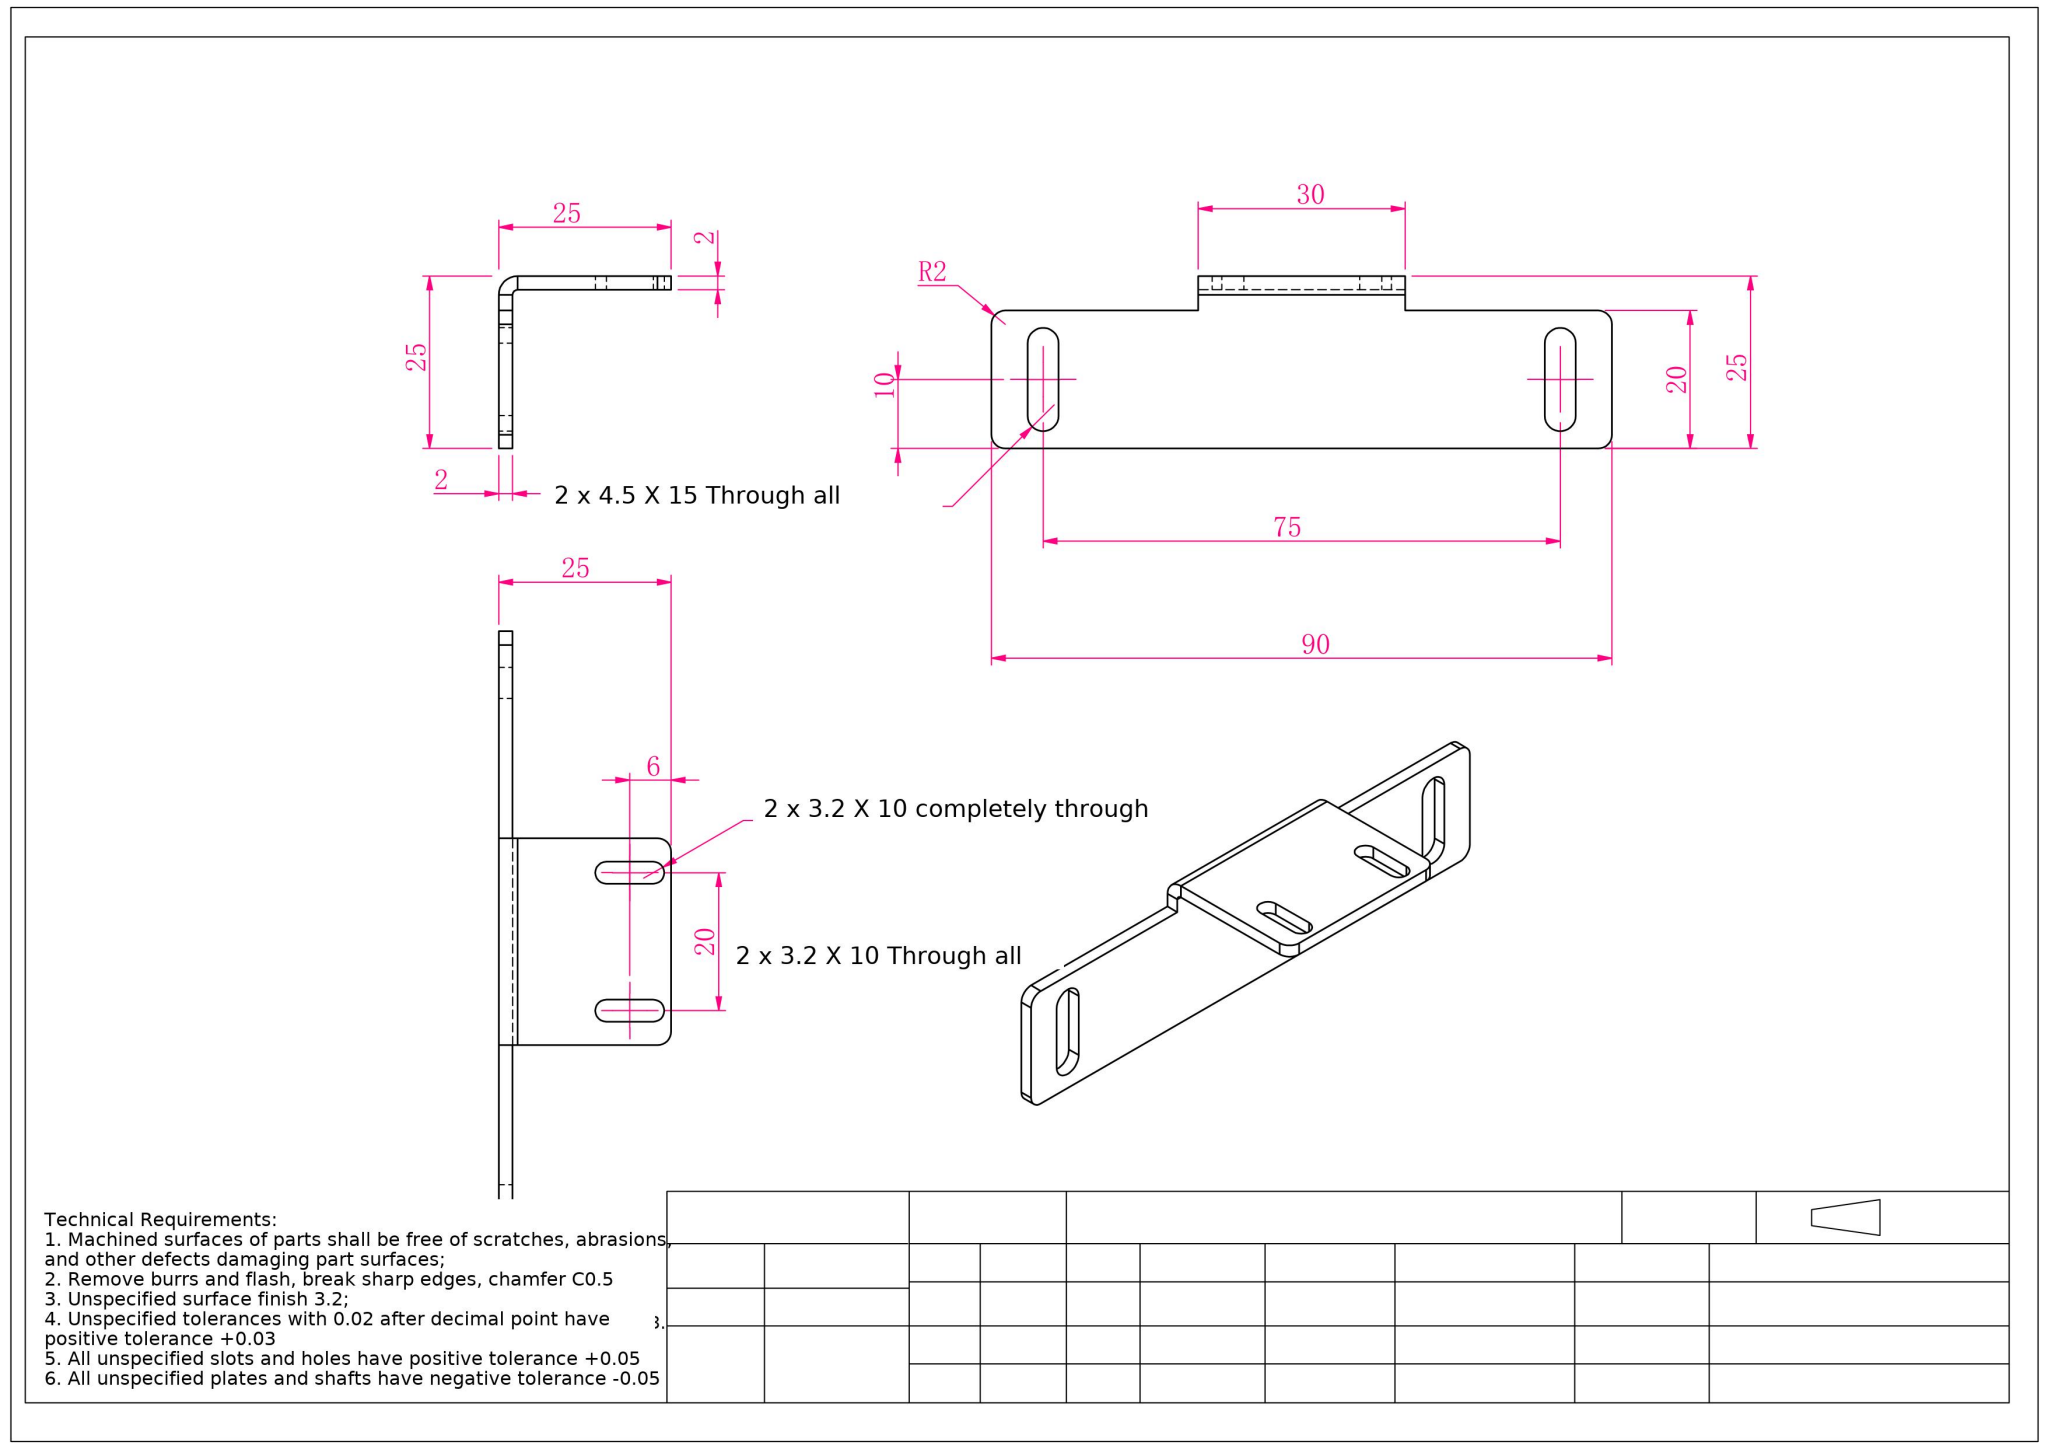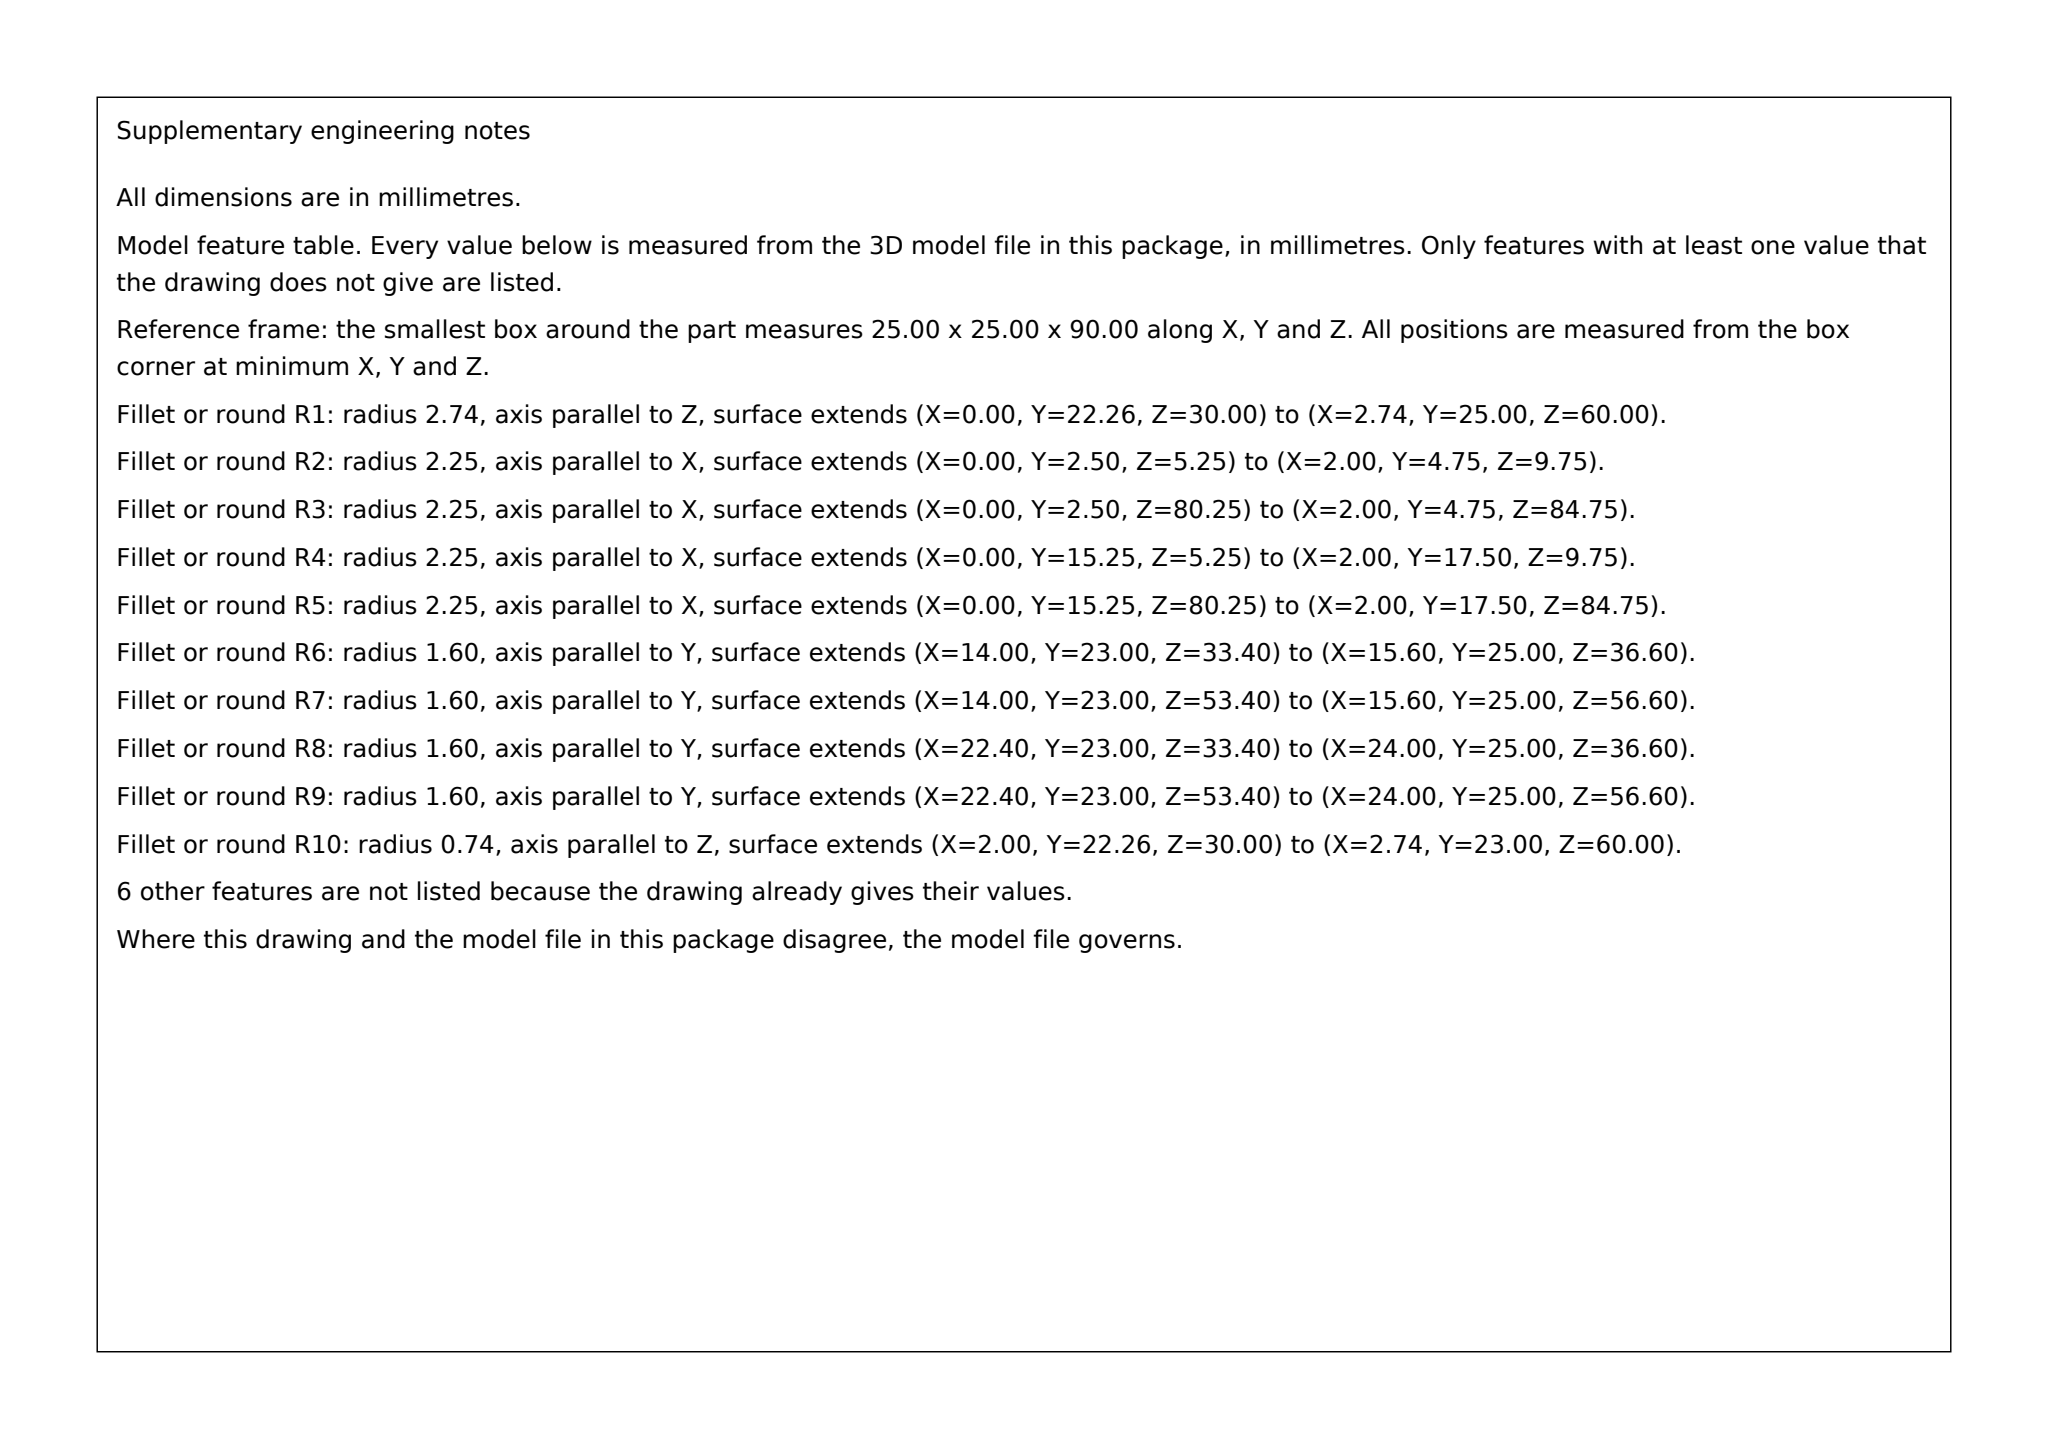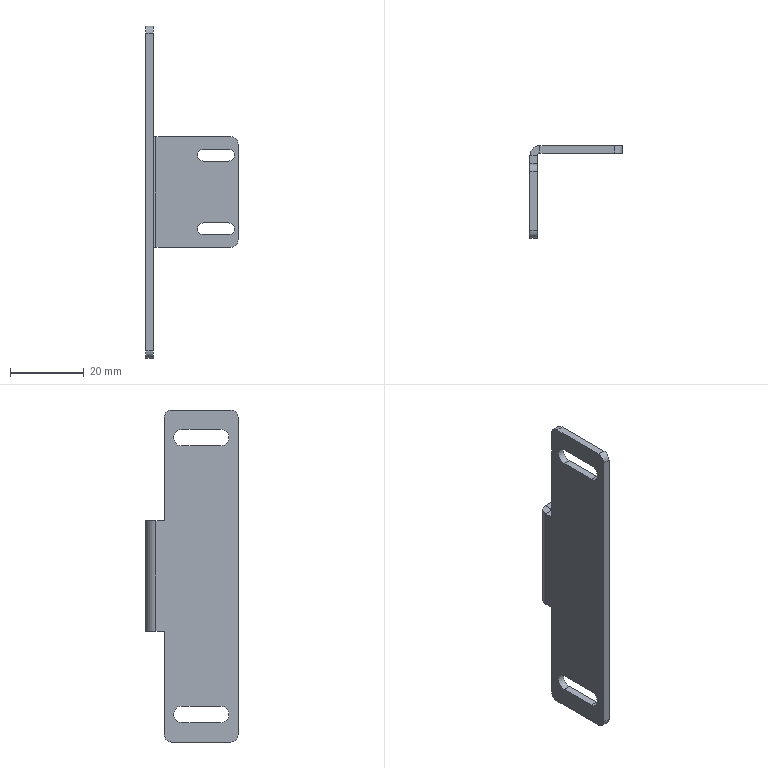Part | SolidWorks | mm | 1 solid | 40 faces | box 25 x 25 x 90 mm | volume 4853 mm3 | plane 24 | cylinder 16 | commonest cylinder face diameters 4 x6 4.5 x4 3.2 x4 5.473 x1 1.473 x1